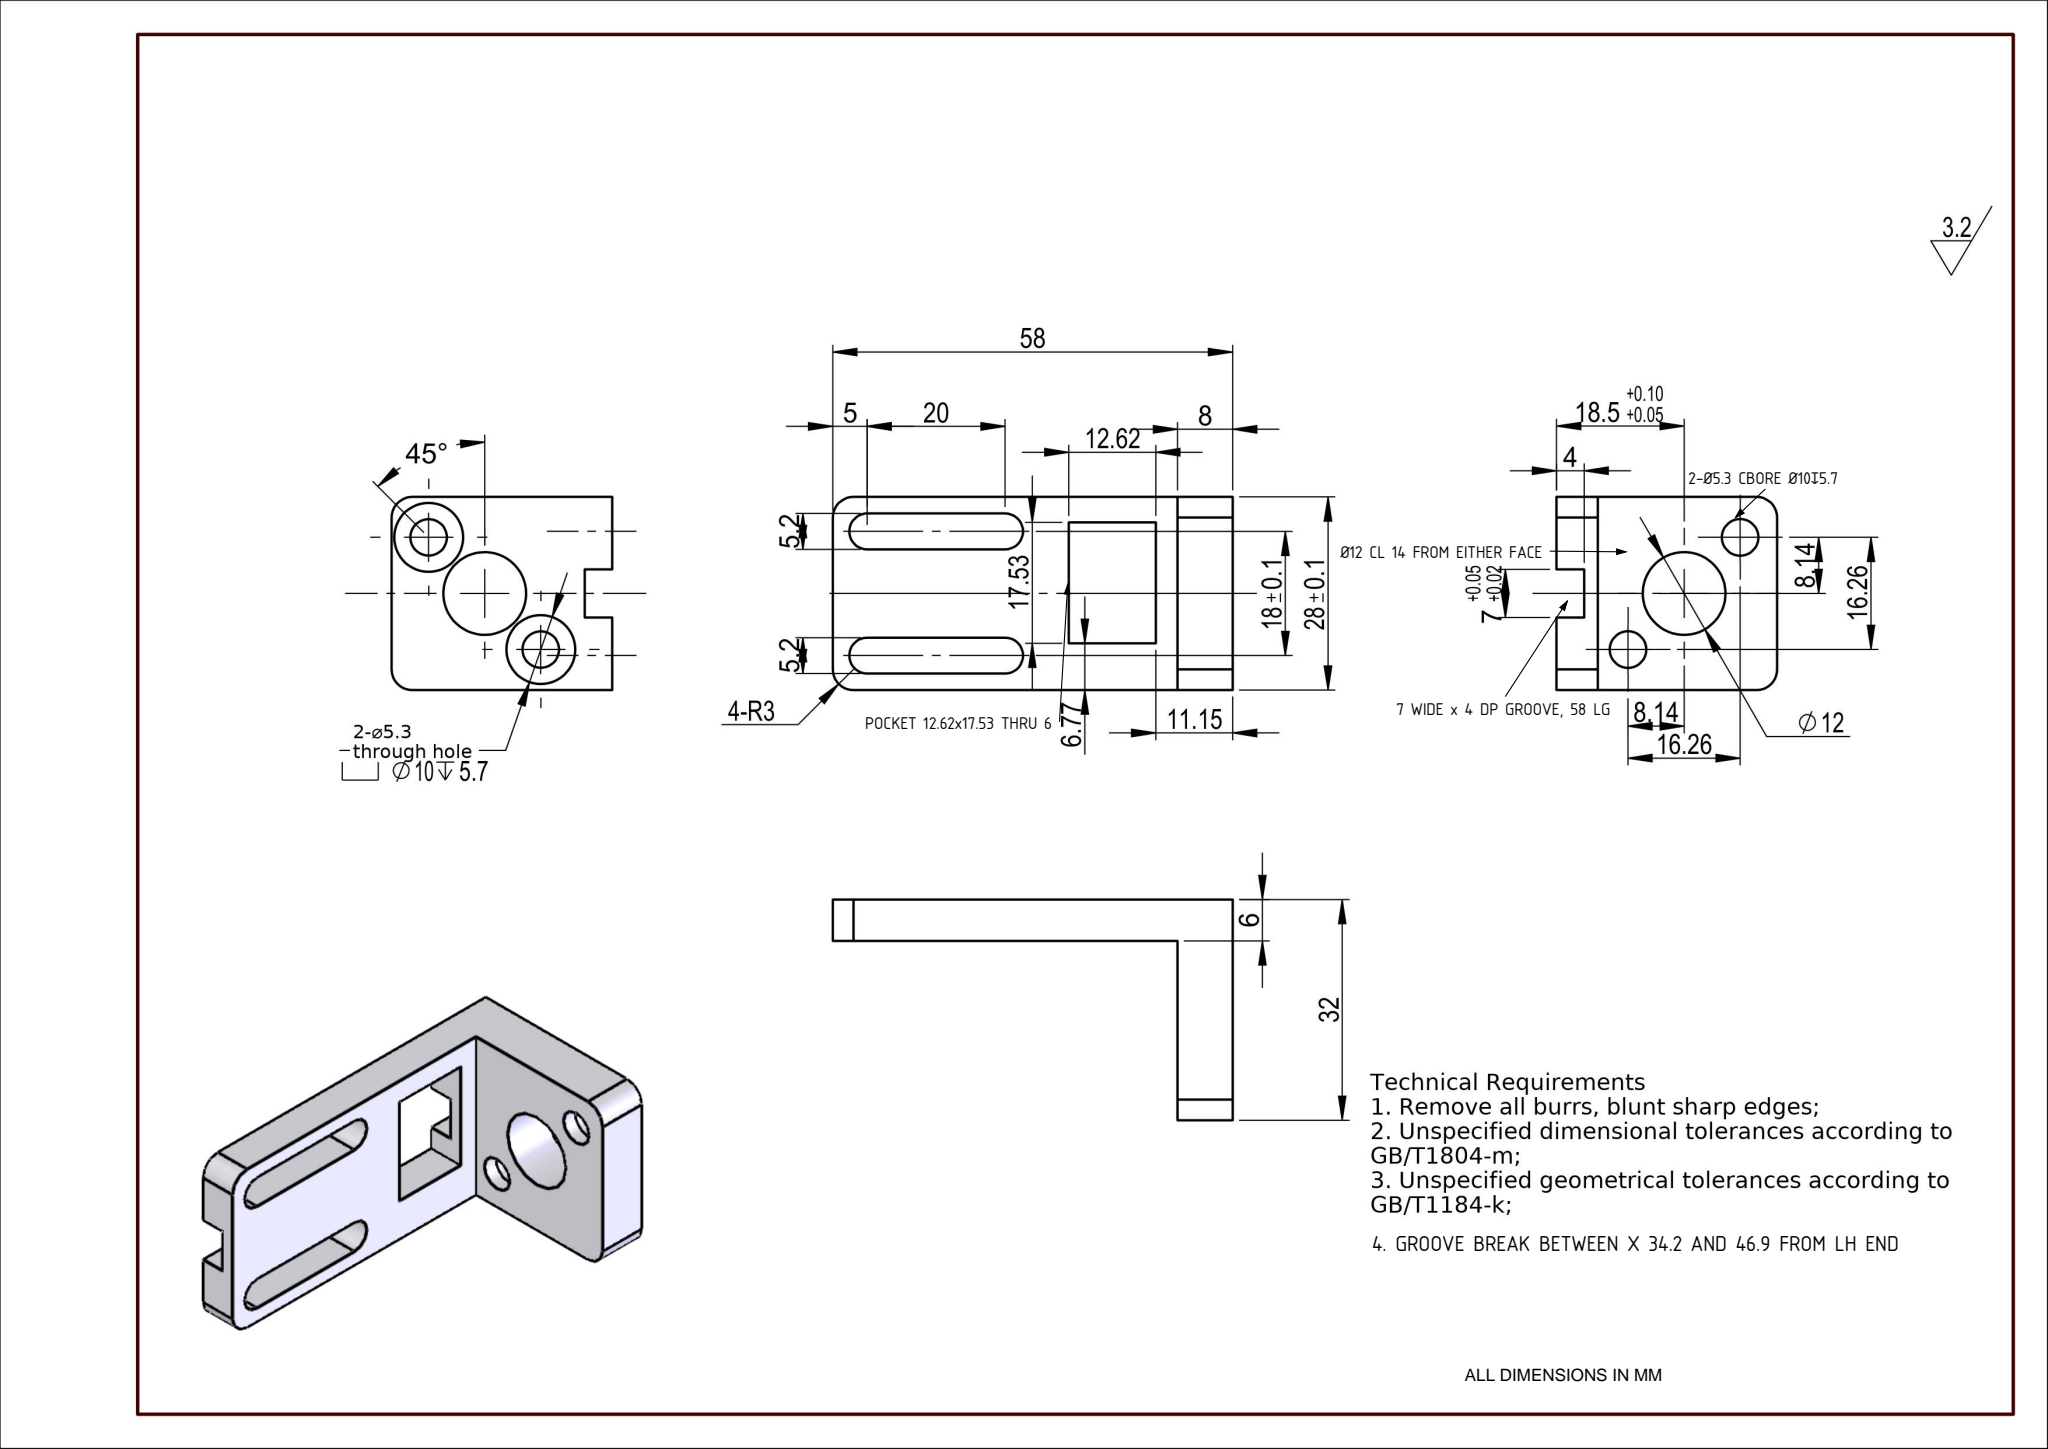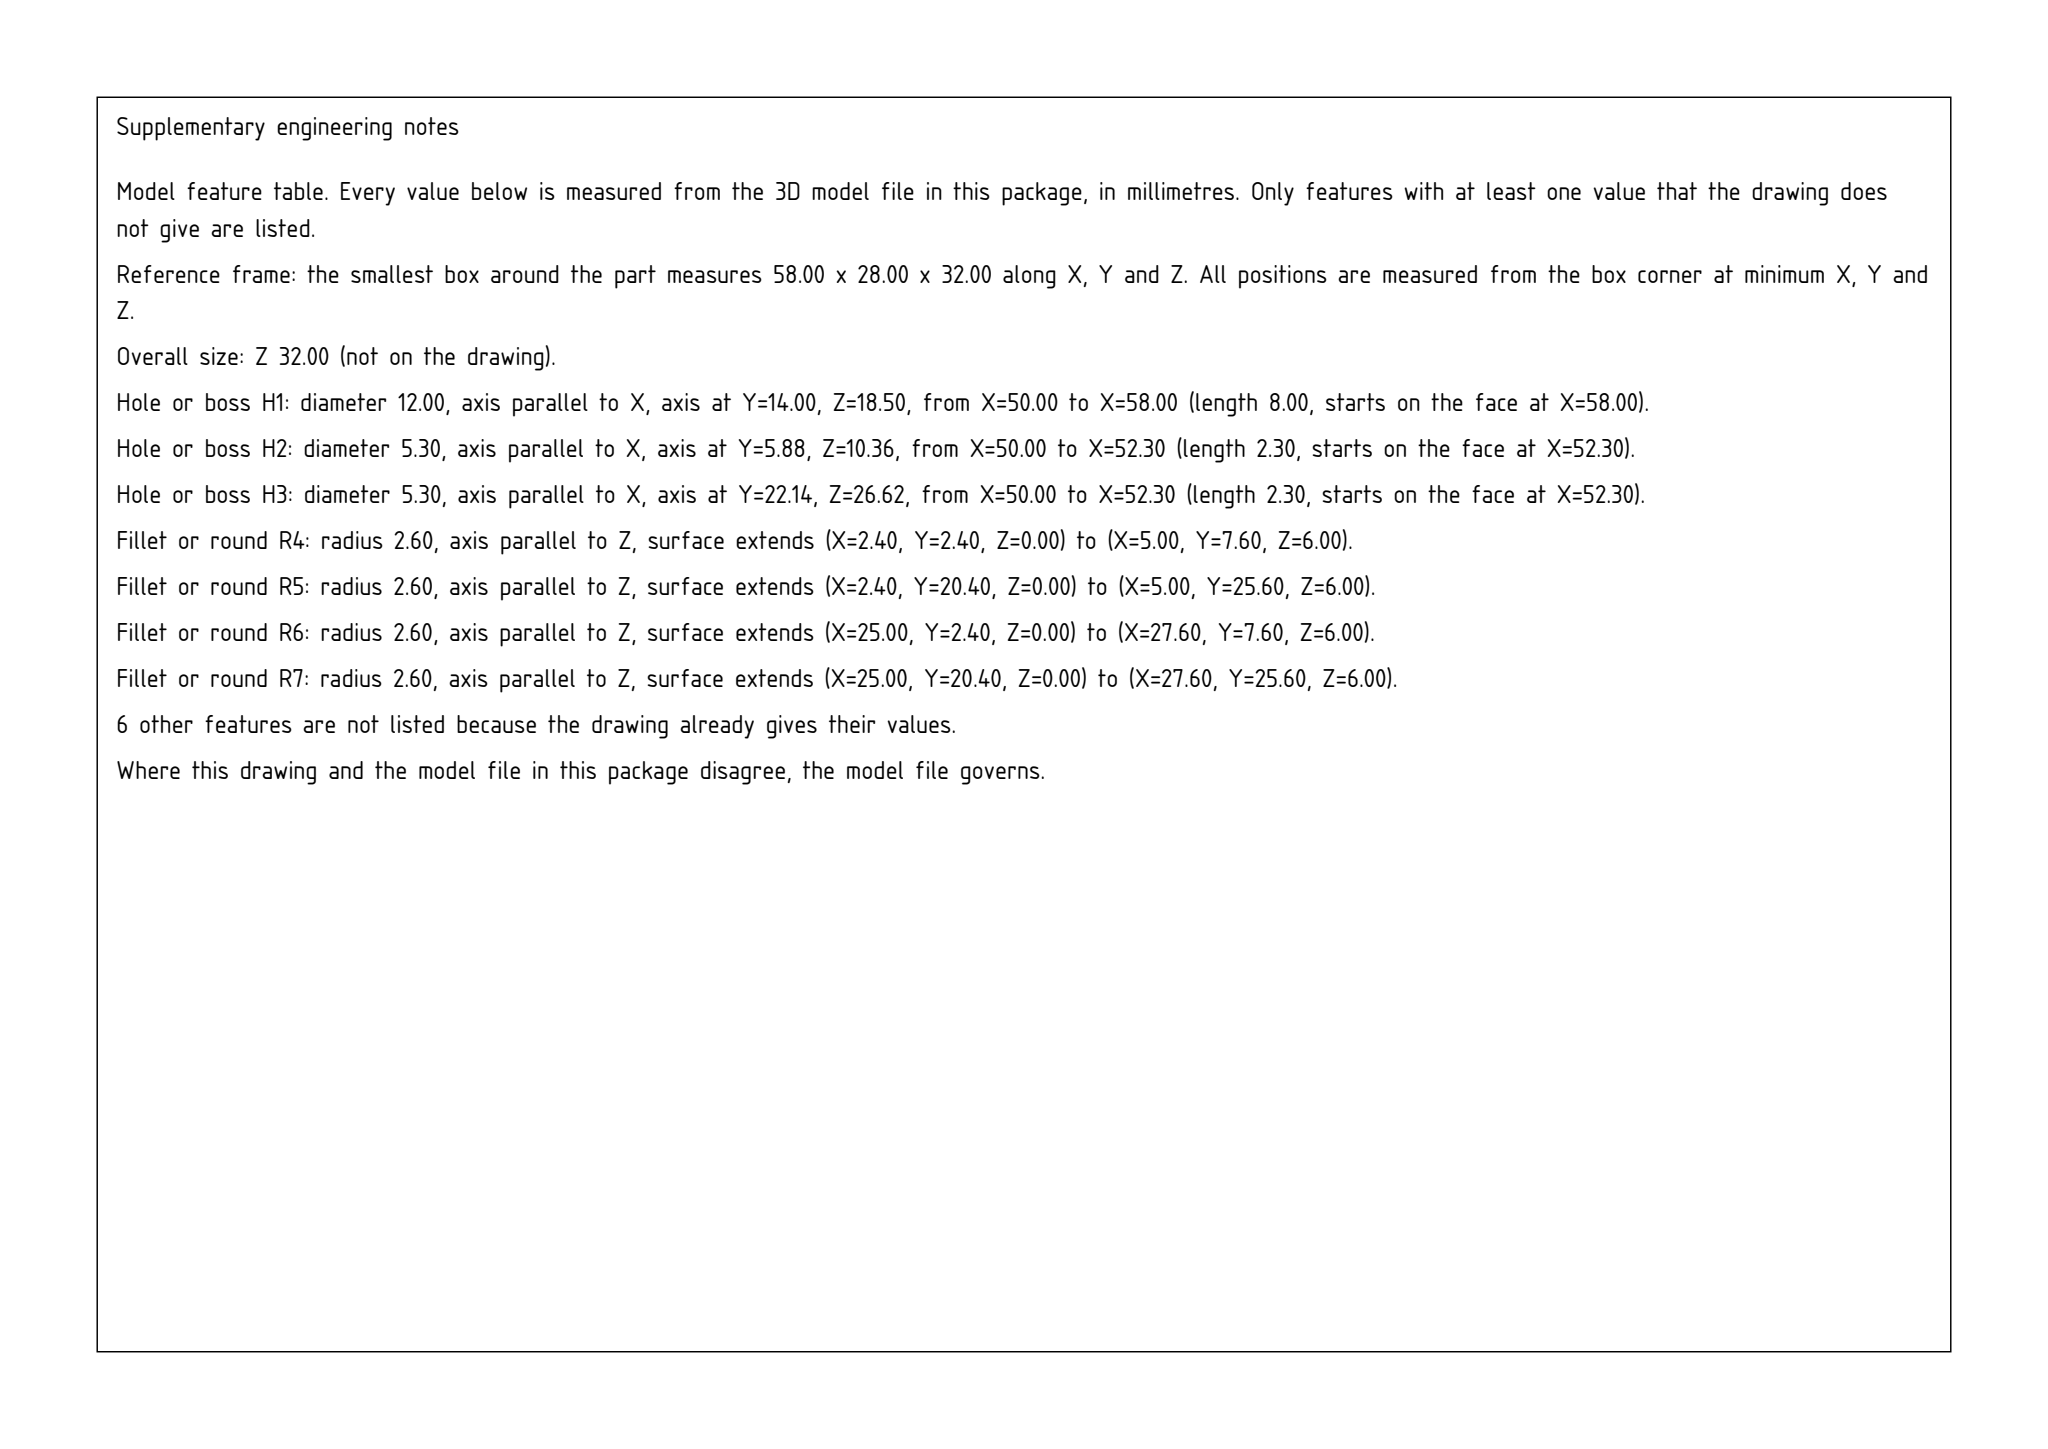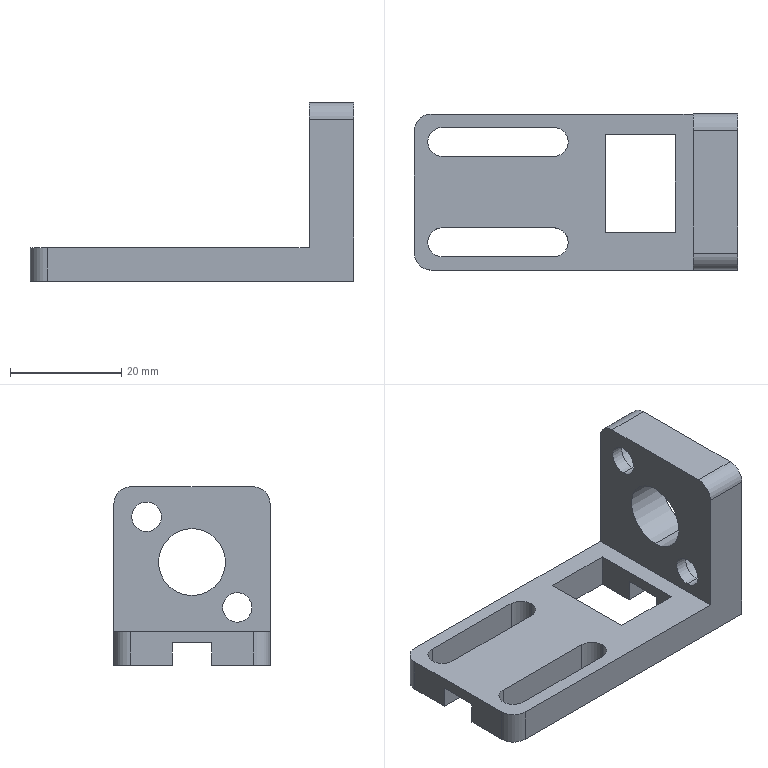Part | SolidWorks | mm | 1 solid | 45 faces | box 58 x 28 x 32 mm | volume 9511 mm3 | plane 25 | cylinder 20 | commonest cylinder face diameters 5.2 x6 10 x4 5.3 x4 6 x4 12 x2
Drawing notes:
POCKET 12.62 x 17.53 THRU 6 THK PLATE | from the solid: Planes x=34.2 & x=46.9 (y 6.8-24.3) and y=6.8 & y=24.3 (x 34.2-46.9) all span z 0-6; no floor face inside pocket, plate thk 6 (z 0-6)
Ø12 BORE CL CENTRED ON 28 WIDTH: 14 FROM EITHER FACE | from the solid: hole/bore dia 12, axis x at [y=14.0, z=18.5]; bbox y 0-28 so CL = 14 = 28/2
2-Ø5.3 C'BORE Ø10 DP 5.7 CL 5.9 & 22.1 FROM 28 EDGE | from the solid: Ø5.3 bores at y=5.9 & 22.1 (z=10.4 & 26.6), x 50.0-52.3; Ø10 c'bore x 52.3-58.0 (5.7 deep)
7 WIDE x 4 DP GROOVE CENTRED ON 28 (CL 14), FULL 58 LG | from the solid: y-planes at 10.5 & 17.5 (7 wide, mid 14), z=4.0 floor, x extents 0-34.2 and 46.9-58.0
GROOVE BREAK BETWEEN X 34.2 AND 46.9 FROM LH END | from the solid: z=4.0 floor planes x[0,34.2] and x[46.9,58.0]; x-planes at 34.2 and 46.9
build123d program:
from build123d import *

# Parameters (mm, degrees)
SKETCH1_W                                            = 58
SKETCH1_H                                            = 28
BOSS_EXTRUDE1_DEPTH                                  = 3
SKETCH2_W                                            = 8
SKETCH2_H                                            = 28
BOSS_EXTRUDE2_DEPTH                                  = 26
SKETCH4_R                                            = 6
CUT_EXTRUDE2_DEPTH                                   = 67.34
CUT_EXTRUDE3_DEPTH                                   = 42.388
SKETCH7_W                                            = 78.454
SKETCH7_H                                            = 7
CUT_EXTRUDE4_DEPTH                                   = 4
HOLE_SIZE_ACCORDING_TO_HEXAGON_SOCKET_HE_D           = 5.3
HOLE_SIZE_ACCORDING_TO_HEXAGON_SOCKET_HE_CBORE_D     = 10
HOLE_SIZE_ACCORDING_TO_HEXAGON_SOCKET_HE_CBORE_DEPTH = 5.7
FILLET1_R                                            = 3
SKETCH10_W                                           = 12.621
SKETCH10_H                                           = 17.531
CUT_EXTRUDE5_DEPTH                                   = 26


with BuildPart() as part:
    # Sketch1 → Boss-Extrude1 (new, symmetric)
    with BuildSketch(Plane.XY):
        Rectangle(SKETCH1_W, SKETCH1_H)
    extrude(amount=BOSS_EXTRUDE1_DEPTH, both=True)

    # Sketch2 → Boss-Extrude2 (add)
    with BuildSketch(Plane.XY.offset(3)):
        with Locations((25, 0)):
            Rectangle(SKETCH2_W, SKETCH2_H)
    extrude(amount=BOSS_EXTRUDE2_DEPTH)

    # Sketch4 → Cut-Extrude2 (cut, through all)
    with BuildSketch(Plane(origin=(29, 0, 0), x_dir=(0, 0, -1), z_dir=(1, 0, 0))):
        with Locations((-15.5, 0)):
            Circle(SKETCH4_R)
    extrude(amount=-CUT_EXTRUDE2_DEPTH, mode=Mode.SUBTRACT)

    # Sketch6 → Cut-Extrude3 (cut, through all)
    with BuildSketch(Plane.XY.offset(3)):
        with BuildLine():
            Line((-24, 11.6), (-4, 11.6))
            ThreePointArc((-4, 11.6), (-1.4, 9), (-4, 6.4))
            Line((-4, 6.4), (-24, 6.4))
            ThreePointArc((-24, 6.4), (-26.6, 9), (-24, 11.6))
        make_face()
        with BuildLine():
            Line((-24, -6.4), (-4, -6.4))
            ThreePointArc((-4, -6.4), (-1.4, -9), (-4, -11.6))
            Line((-4, -11.6), (-24, -11.6))
            ThreePointArc((-24, -11.6), (-26.6, -9), (-24, -6.4))
        make_face()
    extrude(amount=-CUT_EXTRUDE3_DEPTH, mode=Mode.SUBTRACT)

    # Sketch7 → Cut-Extrude4 (cut)
    with BuildSketch(Plane(origin=(0, 0, -3), x_dir=(-1, 0, 0), z_dir=(0, 0, -1))):
        Rectangle(SKETCH7_W, SKETCH7_H)
    extrude(amount=-CUT_EXTRUDE4_DEPTH, mode=Mode.SUBTRACT)

    # Hole Size according to Hexagon Socket He (through all)
    with Locations(Plane(origin=(29, 0, 0), x_dir=(0, 0, -1), z_dir=(1, 0, 0))):
        with Locations((-23.625, 8.139), (-7.361, -8.125)):
            CounterBoreHole(HOLE_SIZE_ACCORDING_TO_HEXAGON_SOCKET_HE_D / 2, HOLE_SIZE_ACCORDING_TO_HEXAGON_SOCKET_HE_CBORE_D / 2, HOLE_SIZE_ACCORDING_TO_HEXAGON_SOCKET_HE_CBORE_DEPTH)

    # Fillet1
    fillet1_edges = [part.edges().sort_by_distance(p)[0] for p in [
        (-29, -14, 0),
        (-29, 14, 0),
        (25, -14, 29),
        (25, 14, 29),
    ]]
    fillet(fillet1_edges, radius=FILLET1_R)

    # Sketch10 → Cut-Extrude5 (cut)
    with BuildSketch(Plane.XY.offset(3)):
        with Locations((11.542, 1.537)):
            Rectangle(SKETCH10_W, SKETCH10_H)
    extrude(amount=-CUT_EXTRUDE5_DEPTH, mode=Mode.SUBTRACT)


solid = part.part